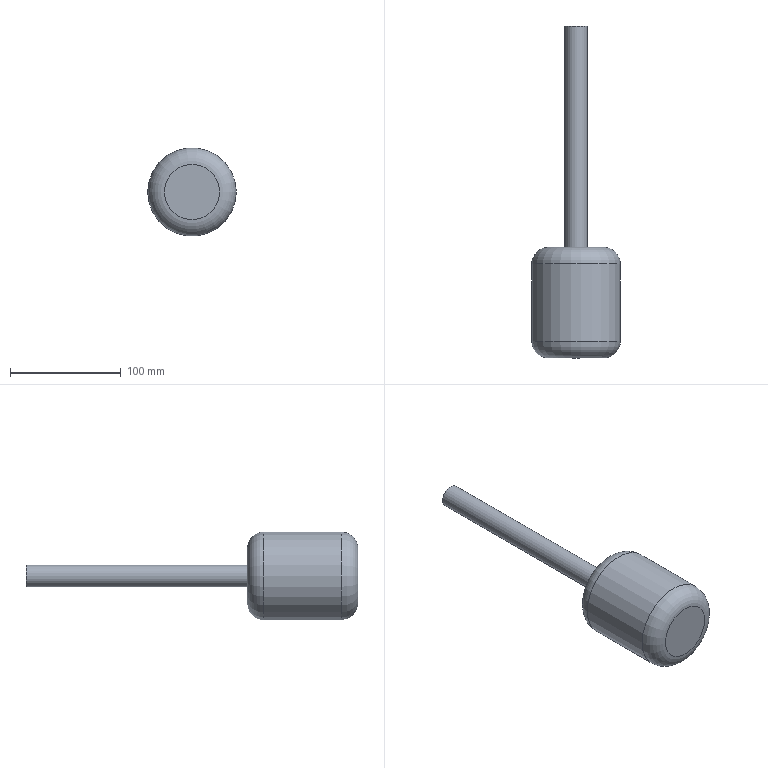Component | NX | MOTOR_ROTOR | 1 solid | 7 faces | box 80 x 300 x 80 mm | volume 543249 mm3 | plane 3 | cylinder 2 | torus 2 | commonest cylinder face diameters 80 x1 20 x1
STEP:
#1=CARTESIAN_POINT('',(0.,0.,0.));
#2=DIRECTION('',(0.,0.,1.));
#3=DIRECTION('',(1.,0.,0.));
#4=AXIS2_PLACEMENT_3D('',#1,#2,#3);
#5=CARTESIAN_POINT('',(-150.,2006.,-0.));
#6=VERTEX_POINT('',#5);
#7=CARTESIAN_POINT('',(-190.,2006.,-0.));
#8=DIRECTION('',(0.,1.,0.));
#9=DIRECTION('',(1.,0.,0.));
#10=AXIS2_PLACEMENT_3D('',#7,#8,#9);
#11=CIRCLE('',#10,40.);
#12=CARTESIAN_POINT('',(-190.,2091.,-0.));
#13=DIRECTION('',(0.,-1.,0.));
#14=DIRECTION('',(-1.,0.,0.));
#15=AXIS2_PLACEMENT_3D('',#12,#13,#14);
#16=CYLINDRICAL_SURFACE('',#15,40.);
#17=CARTESIAN_POINT('',(9.425,85.));
#18=DIRECTION('',(-1.,0.));
#19=VECTOR('',#18,1.);
#20=LINE('',#17,#19);
#21=(GEOMETRIC_REPRESENTATION_CONTEXT(2)PARAMETRIC_REPRESENTATION_CONTEXT()REPRESENTATION_CONTEXT('',''));
#22=DEFINITIONAL_REPRESENTATION('',(#20),#21);
#23=PCURVE('',#16,#22);
#24=CARTESIAN_POINT('',(-190.,2006.,-0.));
#25=DIRECTION('',(0.,1.,0.));
#26=DIRECTION('',(1.,0.,0.));
#27=AXIS2_PLACEMENT_3D('',#24,#25,#26);
#28=TOROIDAL_SURFACE('',#27,25.,15.);
#29=CARTESIAN_POINT('',(0.,6.283));
#30=DIRECTION('',(1.,0.));
#31=VECTOR('',#30,1.);
#32=LINE('',#29,#31);
#33=(GEOMETRIC_REPRESENTATION_CONTEXT(2)PARAMETRIC_REPRESENTATION_CONTEXT()REPRESENTATION_CONTEXT('',''));
#34=DEFINITIONAL_REPRESENTATION('',(#32),#33);
#35=PCURVE('',#28,#34);
#36=SURFACE_CURVE('',#11,(#23,#35),.PCURVE_S1.);
#37=EDGE_CURVE('',#6,#6,#36,.T.);
#38=ORIENTED_EDGE('',*,*,#37,.T.);
#39=CARTESIAN_POINT('',(-150.,2076.,-0.));
#40=VERTEX_POINT('',#39);
#41=CARTESIAN_POINT('',(-150.,2076.,-0.));
#42=CARTESIAN_POINT('',(-150.,2006.,-0.));
#43=B_SPLINE_CURVE_WITH_KNOTS('',1,(#41,#42),.UNSPECIFIED.,.F.,.F.,(2,2),(15.,85.),.PIECEWISE_BEZIER_KNOTS.);
#44=CARTESIAN_POINT('',(3.142,0.));
#45=DIRECTION('',(0.,1.));
#46=VECTOR('',#45,1.);
#47=LINE('',#44,#46);
#48=(GEOMETRIC_REPRESENTATION_CONTEXT(2)PARAMETRIC_REPRESENTATION_CONTEXT()REPRESENTATION_CONTEXT('',''));
#49=DEFINITIONAL_REPRESENTATION('',(#47),#48);
#50=PCURVE('',#16,#49);
#51=CARTESIAN_POINT('',(9.425,0.));
#52=DIRECTION('',(0.,1.));
#53=VECTOR('',#52,1.);
#54=LINE('',#51,#53);
#55=(GEOMETRIC_REPRESENTATION_CONTEXT(2)PARAMETRIC_REPRESENTATION_CONTEXT()REPRESENTATION_CONTEXT('',''));
#56=DEFINITIONAL_REPRESENTATION('',(#54),#55);
#57=PCURVE('',#16,#56);
#58=SEAM_CURVE('',#43,(#50,#57),.PCURVE_S1.);
#59=EDGE_CURVE('',#40,#6,#58,.T.);
#60=ORIENTED_EDGE('',*,*,#59,.F.);
#61=CARTESIAN_POINT('',(-190.,2076.,-0.));
#62=DIRECTION('',(0.,-1.,0.));
#63=DIRECTION('',(1.,0.,0.));
#64=AXIS2_PLACEMENT_3D('',#61,#62,#63);
#65=CIRCLE('',#64,40.);
#66=CARTESIAN_POINT('',(3.142,15.));
#67=DIRECTION('',(1.,0.));
#68=VECTOR('',#67,1.);
#69=LINE('',#66,#68);
#70=(GEOMETRIC_REPRESENTATION_CONTEXT(2)PARAMETRIC_REPRESENTATION_CONTEXT()REPRESENTATION_CONTEXT('',''));
#71=DEFINITIONAL_REPRESENTATION('',(#69),#70);
#72=PCURVE('',#16,#71);
#73=CARTESIAN_POINT('',(-190.,2076.,-0.));
#74=DIRECTION('',(0.,1.,0.));
#75=DIRECTION('',(1.,0.,0.));
#76=AXIS2_PLACEMENT_3D('',#73,#74,#75);
#77=TOROIDAL_SURFACE('',#76,25.,15.);
#78=CARTESIAN_POINT('',(6.283,6.283));
#79=DIRECTION('',(-1.,0.));
#80=VECTOR('',#79,1.);
#81=LINE('',#78,#80);
#82=(GEOMETRIC_REPRESENTATION_CONTEXT(2)PARAMETRIC_REPRESENTATION_CONTEXT()REPRESENTATION_CONTEXT('',''));
#83=DEFINITIONAL_REPRESENTATION('',(#81),#82);
#84=PCURVE('',#77,#83);
#85=SURFACE_CURVE('',#65,(#72,#84),.PCURVE_S1.);
#86=EDGE_CURVE('',#40,#40,#85,.T.);
#87=ORIENTED_EDGE('',*,*,#86,.T.);
#88=ORIENTED_EDGE('',*,*,#59,.T.);
#89=EDGE_LOOP('',(#38,#60,#87,#88));
#90=FACE_BOUND('',#89,.T.);
#91=ADVANCED_FACE('',(#90),#16,.T.);
#92=CARTESIAN_POINT('',(-180.,2091.,-0.));
#93=VERTEX_POINT('',#92);
#94=CARTESIAN_POINT('',(-190.,2091.,-0.));
#95=DIRECTION('',(0.,1.,0.));
#96=DIRECTION('',(1.,0.,0.));
#97=AXIS2_PLACEMENT_3D('',#94,#95,#96);
#98=CIRCLE('',#97,10.);
#99=CARTESIAN_POINT('',(-190.,2091.,-0.));
#100=DIRECTION('',(0.,1.,0.));
#101=DIRECTION('',(1.,0.,0.));
#102=AXIS2_PLACEMENT_3D('',#99,#100,#101);
#103=PLANE('',#102);
#104=CARTESIAN_POINT('',(0.,0.));
#105=DIRECTION('',(1.,0.));
#106=AXIS2_PLACEMENT_2D('',#104,#105);
#107=CIRCLE('',#106,10.);
#108=(GEOMETRIC_REPRESENTATION_CONTEXT(2)PARAMETRIC_REPRESENTATION_CONTEXT()REPRESENTATION_CONTEXT('',''));
#109=DEFINITIONAL_REPRESENTATION('',(#107),#108);
#110=PCURVE('',#103,#109);
#111=CARTESIAN_POINT('',(-190.,2091.,-0.));
#112=DIRECTION('',(0.,1.,0.));
#113=DIRECTION('',(1.,0.,0.));
#114=AXIS2_PLACEMENT_3D('',#111,#112,#113);
#115=CYLINDRICAL_SURFACE('',#114,10.);
#116=CARTESIAN_POINT('',(0.,0.));
#117=DIRECTION('',(1.,0.));
#118=VECTOR('',#117,1.);
#119=LINE('',#116,#118);
#120=(GEOMETRIC_REPRESENTATION_CONTEXT(2)PARAMETRIC_REPRESENTATION_CONTEXT()REPRESENTATION_CONTEXT('',''));
#121=DEFINITIONAL_REPRESENTATION('',(#119),#120);
#122=PCURVE('',#115,#121);
#123=SURFACE_CURVE('',#98,(#110,#122),.PCURVE_S1.);
#124=EDGE_CURVE('',#93,#93,#123,.T.);
#125=ORIENTED_EDGE('',*,*,#124,.F.);
#126=EDGE_LOOP('',(#125));
#127=FACE_BOUND('',#126,.T.);
#128=CARTESIAN_POINT('',(-165.,2091.,-0.));
#129=VERTEX_POINT('',#128);
#130=CARTESIAN_POINT('',(-190.,2091.,-0.));
#131=DIRECTION('',(0.,1.,0.));
#132=DIRECTION('',(1.,0.,0.));
#133=AXIS2_PLACEMENT_3D('',#130,#131,#132);
#134=CIRCLE('',#133,25.);
#135=CARTESIAN_POINT('',(0.,0.));
#136=DIRECTION('',(1.,0.));
#137=AXIS2_PLACEMENT_2D('',#135,#136);
#138=CIRCLE('',#137,25.);
#139=(GEOMETRIC_REPRESENTATION_CONTEXT(2)PARAMETRIC_REPRESENTATION_CONTEXT()REPRESENTATION_CONTEXT('',''));
#140=DEFINITIONAL_REPRESENTATION('',(#138),#139);
#141=PCURVE('',#103,#140);
#142=CARTESIAN_POINT('',(0.,7.854));
#143=DIRECTION('',(1.,0.));
#144=VECTOR('',#143,1.);
#145=LINE('',#142,#144);
#146=(GEOMETRIC_REPRESENTATION_CONTEXT(2)PARAMETRIC_REPRESENTATION_CONTEXT()REPRESENTATION_CONTEXT('',''));
#147=DEFINITIONAL_REPRESENTATION('',(#145),#146);
#148=PCURVE('',#77,#147);
#149=SURFACE_CURVE('',#134,(#141,#148),.PCURVE_S1.);
#150=EDGE_CURVE('',#129,#129,#149,.T.);
#151=ORIENTED_EDGE('',*,*,#150,.T.);
#152=EDGE_LOOP('',(#151));
#153=FACE_BOUND('',#152,.T.);
#154=ADVANCED_FACE('',(#127,#153),#103,.T.);
#155=CARTESIAN_POINT('',(-165.,1991.,-0.));
#156=VERTEX_POINT('',#155);
#157=CARTESIAN_POINT('',(-190.,1991.,-0.));
#158=DIRECTION('',(0.,-1.,0.));
#159=DIRECTION('',(1.,0.,0.));
#160=AXIS2_PLACEMENT_3D('',#157,#158,#159);
#161=CIRCLE('',#160,25.);
#162=CARTESIAN_POINT('',(-190.,1991.,-0.));
#163=DIRECTION('',(0.,1.,0.));
#164=DIRECTION('',(1.,0.,0.));
#165=AXIS2_PLACEMENT_3D('',#162,#163,#164);
#166=PLANE('',#165);
#167=CARTESIAN_POINT('',(25.,0.));
#168=CARTESIAN_POINT('',(25.,-43.301));
#169=CARTESIAN_POINT('',(-12.5,-21.651));
#170=CARTESIAN_POINT('',(-50.,-0.));
#171=CARTESIAN_POINT('',(-12.5,21.651));
#172=CARTESIAN_POINT('',(25.,43.301));
#173=CARTESIAN_POINT('',(25.,0.));
#174=(BOUNDED_CURVE()B_SPLINE_CURVE(2,(#167,#168,#169,#170,#171,#172,#173),.UNSPECIFIED.,.T.,.F.)B_SPLINE_CURVE_WITH_KNOTS((1,2,2,2,2,1),(-2.094,0.,2.094,4.189,6.283,8.378),.UNSPECIFIED.)CURVE()GEOMETRIC_REPRESENTATION_ITEM()RATIONAL_B_SPLINE_CURVE((1.,0.5,1.,0.5,1.,0.5,1.))REPRESENTATION_ITEM(''));
#175=(GEOMETRIC_REPRESENTATION_CONTEXT(2)PARAMETRIC_REPRESENTATION_CONTEXT()REPRESENTATION_CONTEXT('',''));
#176=DEFINITIONAL_REPRESENTATION('',(#174),#175);
#177=PCURVE('',#166,#176);
#178=CARTESIAN_POINT('',(6.283,4.712));
#179=DIRECTION('',(-1.,0.));
#180=VECTOR('',#179,1.);
#181=LINE('',#178,#180);
#182=(GEOMETRIC_REPRESENTATION_CONTEXT(2)PARAMETRIC_REPRESENTATION_CONTEXT()REPRESENTATION_CONTEXT('',''));
#183=DEFINITIONAL_REPRESENTATION('',(#181),#182);
#184=PCURVE('',#28,#183);
#185=SURFACE_CURVE('',#161,(#177,#184),.PCURVE_S1.);
#186=EDGE_CURVE('',#156,#156,#185,.T.);
#187=ORIENTED_EDGE('',*,*,#186,.T.);
#188=EDGE_LOOP('',(#187));
#189=FACE_BOUND('',#188,.T.);
#190=ADVANCED_FACE('',(#189),#166,.F.);
#191=ORIENTED_EDGE('',*,*,#186,.F.);
#192=CARTESIAN_POINT('',(-165.,1991.,-0.));
#193=CARTESIAN_POINT('',(-160.99,1991.,-0.));
#194=CARTESIAN_POINT('',(-157.084,1992.275,-0.));
#195=CARTESIAN_POINT('',(-153.721,1994.721,-0.));
#196=CARTESIAN_POINT('',(-151.275,1998.084,-0.));
#197=CARTESIAN_POINT('',(-150.,2001.99,-0.));
#198=CARTESIAN_POINT('',(-150.,2006.,-0.));
#199=(BOUNDED_CURVE()B_SPLINE_CURVE(6,(#192,#193,#194,#195,#196,#197,#198),.UNSPECIFIED.,.F.,.F.)B_SPLINE_CURVE_WITH_KNOTS((7,7),(4.712,6.283),.PIECEWISE_BEZIER_KNOTS.)CURVE()GEOMETRIC_REPRESENTATION_ITEM()RATIONAL_B_SPLINE_CURVE((1.031,1.01,0.9979,0.994,0.9979,1.01,1.031))REPRESENTATION_ITEM(''));
#200=CARTESIAN_POINT('',(6.283,0.));
#201=DIRECTION('',(0.,1.));
#202=VECTOR('',#201,1.);
#203=LINE('',#200,#202);
#204=(GEOMETRIC_REPRESENTATION_CONTEXT(2)PARAMETRIC_REPRESENTATION_CONTEXT()REPRESENTATION_CONTEXT('',''));
#205=DEFINITIONAL_REPRESENTATION('',(#203),#204);
#206=PCURVE('',#28,#205);
#207=CARTESIAN_POINT('',(0.,0.));
#208=DIRECTION('',(0.,1.));
#209=VECTOR('',#208,1.);
#210=LINE('',#207,#209);
#211=(GEOMETRIC_REPRESENTATION_CONTEXT(2)PARAMETRIC_REPRESENTATION_CONTEXT()REPRESENTATION_CONTEXT('',''));
#212=DEFINITIONAL_REPRESENTATION('',(#210),#211);
#213=PCURVE('',#28,#212);
#214=SEAM_CURVE('',#199,(#206,#213),.PCURVE_S1.);
#215=EDGE_CURVE('',#156,#6,#214,.T.);
#216=ORIENTED_EDGE('',*,*,#215,.T.);
#217=ORIENTED_EDGE('',*,*,#37,.F.);
#218=ORIENTED_EDGE('',*,*,#215,.F.);
#219=EDGE_LOOP('',(#191,#216,#217,#218));
#220=FACE_BOUND('',#219,.T.);
#221=ADVANCED_FACE('',(#220),#28,.T.);
#222=ORIENTED_EDGE('',*,*,#86,.F.);
#223=CARTESIAN_POINT('',(-150.,2076.,-0.));
#224=CARTESIAN_POINT('',(-150.,2080.01,-0.));
#225=CARTESIAN_POINT('',(-151.275,2083.916,-0.));
#226=CARTESIAN_POINT('',(-153.721,2087.279,-0.));
#227=CARTESIAN_POINT('',(-157.084,2089.725,-0.));
#228=CARTESIAN_POINT('',(-160.99,2091.,-0.));
#229=CARTESIAN_POINT('',(-165.,2091.,-0.));
#230=(BOUNDED_CURVE()B_SPLINE_CURVE(6,(#223,#224,#225,#226,#227,#228,#229),.UNSPECIFIED.,.F.,.F.)B_SPLINE_CURVE_WITH_KNOTS((7,7),(0.,1.571),.PIECEWISE_BEZIER_KNOTS.)CURVE()GEOMETRIC_REPRESENTATION_ITEM()RATIONAL_B_SPLINE_CURVE((1.031,1.01,0.9979,0.994,0.9979,1.01,1.031))REPRESENTATION_ITEM(''));
#231=CARTESIAN_POINT('',(6.283,6.283));
#232=DIRECTION('',(0.,1.));
#233=VECTOR('',#232,1.);
#234=LINE('',#231,#233);
#235=(GEOMETRIC_REPRESENTATION_CONTEXT(2)PARAMETRIC_REPRESENTATION_CONTEXT()REPRESENTATION_CONTEXT('',''));
#236=DEFINITIONAL_REPRESENTATION('',(#234),#235);
#237=PCURVE('',#77,#236);
#238=CARTESIAN_POINT('',(0.,6.283));
#239=DIRECTION('',(0.,1.));
#240=VECTOR('',#239,1.);
#241=LINE('',#238,#240);
#242=(GEOMETRIC_REPRESENTATION_CONTEXT(2)PARAMETRIC_REPRESENTATION_CONTEXT()REPRESENTATION_CONTEXT('',''));
#243=DEFINITIONAL_REPRESENTATION('',(#241),#242);
#244=PCURVE('',#77,#243);
#245=SEAM_CURVE('',#230,(#237,#244),.PCURVE_S1.);
#246=EDGE_CURVE('',#40,#129,#245,.T.);
#247=ORIENTED_EDGE('',*,*,#246,.T.);
#248=ORIENTED_EDGE('',*,*,#150,.F.);
#249=ORIENTED_EDGE('',*,*,#246,.F.);
#250=EDGE_LOOP('',(#222,#247,#248,#249));
#251=FACE_BOUND('',#250,.T.);
#252=ADVANCED_FACE('',(#251),#77,.T.);
#253=CARTESIAN_POINT('',(-180.,2291.,-0.));
#254=VERTEX_POINT('',#253);
#255=CARTESIAN_POINT('',(-190.,2291.,-0.));
#256=DIRECTION('',(0.,-1.,0.));
#257=DIRECTION('',(1.,0.,0.));
#258=AXIS2_PLACEMENT_3D('',#255,#256,#257);
#259=CIRCLE('',#258,10.);
#260=CARTESIAN_POINT('',(-190.,2291.,-0.));
#261=DIRECTION('',(0.,1.,0.));
#262=DIRECTION('',(1.,0.,0.));
#263=AXIS2_PLACEMENT_3D('',#260,#261,#262);
#264=PLANE('',#263);
#265=CARTESIAN_POINT('',(10.,0.));
#266=CARTESIAN_POINT('',(10.,-17.321));
#267=CARTESIAN_POINT('',(-5.,-8.66));
#268=CARTESIAN_POINT('',(-20.,-0.));
#269=CARTESIAN_POINT('',(-5.,8.66));
#270=CARTESIAN_POINT('',(10.,17.321));
#271=CARTESIAN_POINT('',(10.,0.));
#272=(BOUNDED_CURVE()B_SPLINE_CURVE(2,(#265,#266,#267,#268,#269,#270,#271),.UNSPECIFIED.,.T.,.F.)B_SPLINE_CURVE_WITH_KNOTS((1,2,2,2,2,1),(-2.094,0.,2.094,4.189,6.283,8.378),.UNSPECIFIED.)CURVE()GEOMETRIC_REPRESENTATION_ITEM()RATIONAL_B_SPLINE_CURVE((1.,0.5,1.,0.5,1.,0.5,1.))REPRESENTATION_ITEM(''));
#273=(GEOMETRIC_REPRESENTATION_CONTEXT(2)PARAMETRIC_REPRESENTATION_CONTEXT()REPRESENTATION_CONTEXT('',''));
#274=DEFINITIONAL_REPRESENTATION('',(#272),#273);
#275=PCURVE('',#264,#274);
#276=CARTESIAN_POINT('',(6.283,200.));
#277=DIRECTION('',(-1.,0.));
#278=VECTOR('',#277,1.);
#279=LINE('',#276,#278);
#280=(GEOMETRIC_REPRESENTATION_CONTEXT(2)PARAMETRIC_REPRESENTATION_CONTEXT()REPRESENTATION_CONTEXT('',''));
#281=DEFINITIONAL_REPRESENTATION('',(#279),#280);
#282=PCURVE('',#115,#281);
#283=SURFACE_CURVE('',#259,(#275,#282),.PCURVE_S1.);
#284=EDGE_CURVE('',#254,#254,#283,.T.);
#285=ORIENTED_EDGE('',*,*,#284,.F.);
#286=EDGE_LOOP('',(#285));
#287=FACE_BOUND('',#286,.T.);
#288=ADVANCED_FACE('',(#287),#264,.T.);
#289=ORIENTED_EDGE('',*,*,#284,.T.);
#290=CARTESIAN_POINT('',(-180.,2091.,-0.));
#291=CARTESIAN_POINT('',(-180.,2291.,-0.));
#292=B_SPLINE_CURVE_WITH_KNOTS('',1,(#290,#291),.UNSPECIFIED.,.F.,.F.,(2,2),(0.,200.),.PIECEWISE_BEZIER_KNOTS.);
#293=CARTESIAN_POINT('',(0.,0.));
#294=DIRECTION('',(0.,1.));
#295=VECTOR('',#294,1.);
#296=LINE('',#293,#295);
#297=(GEOMETRIC_REPRESENTATION_CONTEXT(2)PARAMETRIC_REPRESENTATION_CONTEXT()REPRESENTATION_CONTEXT('',''));
#298=DEFINITIONAL_REPRESENTATION('',(#296),#297);
#299=PCURVE('',#115,#298);
#300=CARTESIAN_POINT('',(6.283,0.));
#301=DIRECTION('',(0.,1.));
#302=VECTOR('',#301,1.);
#303=LINE('',#300,#302);
#304=(GEOMETRIC_REPRESENTATION_CONTEXT(2)PARAMETRIC_REPRESENTATION_CONTEXT()REPRESENTATION_CONTEXT('',''));
#305=DEFINITIONAL_REPRESENTATION('',(#303),#304);
#306=PCURVE('',#115,#305);
#307=SEAM_CURVE('',#292,(#299,#306),.PCURVE_S1.);
#308=EDGE_CURVE('',#93,#254,#307,.T.);
#309=ORIENTED_EDGE('',*,*,#308,.F.);
#310=ORIENTED_EDGE('',*,*,#124,.T.);
#311=ORIENTED_EDGE('',*,*,#308,.T.);
#312=EDGE_LOOP('',(#289,#309,#310,#311));
#313=FACE_BOUND('',#312,.T.);
#314=ADVANCED_FACE('',(#313),#115,.T.);
#315=CLOSED_SHELL('',(#91,#154,#190,#221,#252,#288,#314));
#316=MANIFOLD_SOLID_BREP('',#315);
#317=(LENGTH_UNIT()NAMED_UNIT(*)SI_UNIT(.MILLI.,.METRE.));
#318=UNCERTAINTY_MEASURE_WITH_UNIT(LENGTH_MEASURE(0.00001),#317,'','');
#319=(NAMED_UNIT(*)PLANE_ANGLE_UNIT()SI_UNIT($,.RADIAN.));
#320=(NAMED_UNIT(*)SI_UNIT($,.STERADIAN.)SOLID_ANGLE_UNIT());
#321=(GEOMETRIC_REPRESENTATION_CONTEXT(3)GLOBAL_UNCERTAINTY_ASSIGNED_CONTEXT((#318))GLOBAL_UNIT_ASSIGNED_CONTEXT((#317,#319,#320))REPRESENTATION_CONTEXT('',''));
#322=ADVANCED_BREP_SHAPE_REPRESENTATION('',(#4,#316),#321);